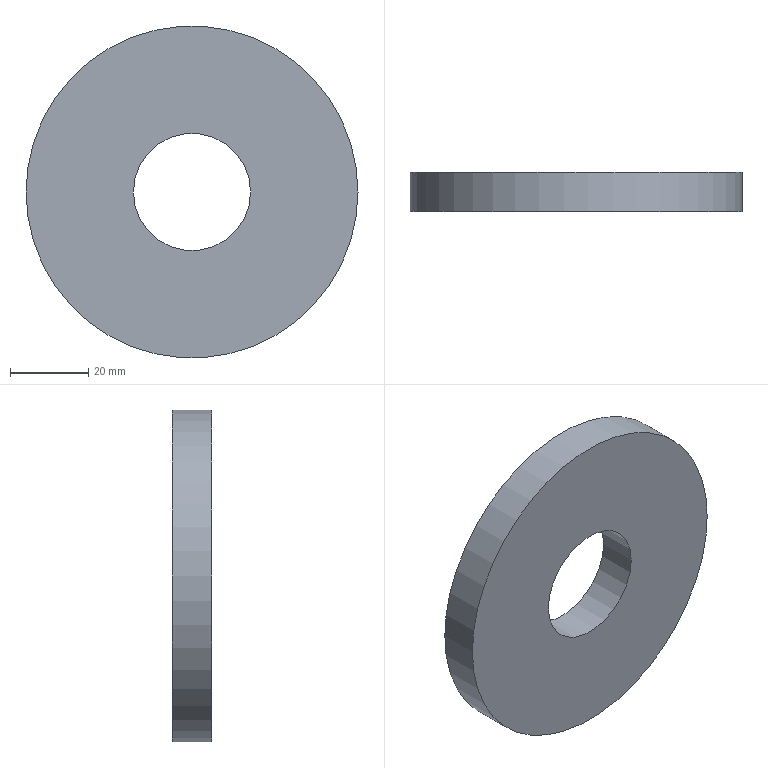Component | NX | SWASH_PLATE | 1 solid | 4 faces | box 85 x 10 x 85 mm | volume 49676 mm3 | cylinder 2 | plane 2 | commonest cylinder face diameters 85 x1 30 x1
STEP:
#1=CARTESIAN_POINT('',(0.,0.,0.));
#2=DIRECTION('',(0.,0.,1.));
#3=DIRECTION('',(1.,0.,0.));
#4=AXIS2_PLACEMENT_3D('',#1,#2,#3);
#5=CARTESIAN_POINT('',(42.5,99.,-0.));
#6=VERTEX_POINT('',#5);
#7=CARTESIAN_POINT('',(0.,99.,-0.));
#8=DIRECTION('',(0.,-1.,0.));
#9=DIRECTION('',(1.,0.,-0.));
#10=AXIS2_PLACEMENT_3D('',#7,#8,#9);
#11=CIRCLE('',#10,42.5);
#12=CARTESIAN_POINT('',(0.,99.,-0.));
#13=DIRECTION('',(0.,1.,0.));
#14=DIRECTION('',(0.,0.,1.));
#15=AXIS2_PLACEMENT_3D('',#12,#13,#14);
#16=CYLINDRICAL_SURFACE('',#15,42.5);
#17=CARTESIAN_POINT('',(7.854,0.));
#18=DIRECTION('',(-1.,0.));
#19=VECTOR('',#18,1.);
#20=LINE('',#17,#19);
#21=(GEOMETRIC_REPRESENTATION_CONTEXT(2)PARAMETRIC_REPRESENTATION_CONTEXT()REPRESENTATION_CONTEXT('',''));
#22=DEFINITIONAL_REPRESENTATION('',(#20),#21);
#23=PCURVE('',#16,#22);
#24=CARTESIAN_POINT('',(0.,99.,-0.));
#25=DIRECTION('',(0.,-1.,0.));
#26=DIRECTION('',(0.,0.,-1.));
#27=AXIS2_PLACEMENT_3D('',#24,#25,#26);
#28=PLANE('',#27);
#29=CARTESIAN_POINT('',(0.,0.));
#30=DIRECTION('',(0.,1.));
#31=AXIS2_PLACEMENT_2D('',#29,#30);
#32=CIRCLE('',#31,42.5);
#33=(GEOMETRIC_REPRESENTATION_CONTEXT(2)PARAMETRIC_REPRESENTATION_CONTEXT()REPRESENTATION_CONTEXT('',''));
#34=DEFINITIONAL_REPRESENTATION('',(#32),#33);
#35=PCURVE('',#28,#34);
#36=SURFACE_CURVE('',#11,(#23,#35),.PCURVE_S1.);
#37=EDGE_CURVE('',#6,#6,#36,.T.);
#38=ORIENTED_EDGE('',*,*,#37,.F.);
#39=CARTESIAN_POINT('',(42.5,109.,-0.));
#40=VERTEX_POINT('',#39);
#41=CARTESIAN_POINT('',(42.5,99.,-0.));
#42=CARTESIAN_POINT('',(42.5,109.,-0.));
#43=B_SPLINE_CURVE_WITH_KNOTS('',1,(#41,#42),.UNSPECIFIED.,.F.,.F.,(2,2),(0.,10.),.PIECEWISE_BEZIER_KNOTS.);
#44=CARTESIAN_POINT('',(7.854,0.));
#45=DIRECTION('',(0.,1.));
#46=VECTOR('',#45,1.);
#47=LINE('',#44,#46);
#48=(GEOMETRIC_REPRESENTATION_CONTEXT(2)PARAMETRIC_REPRESENTATION_CONTEXT()REPRESENTATION_CONTEXT('',''));
#49=DEFINITIONAL_REPRESENTATION('',(#47),#48);
#50=PCURVE('',#16,#49);
#51=CARTESIAN_POINT('',(1.571,0.));
#52=DIRECTION('',(0.,1.));
#53=VECTOR('',#52,1.);
#54=LINE('',#51,#53);
#55=(GEOMETRIC_REPRESENTATION_CONTEXT(2)PARAMETRIC_REPRESENTATION_CONTEXT()REPRESENTATION_CONTEXT('',''));
#56=DEFINITIONAL_REPRESENTATION('',(#54),#55);
#57=PCURVE('',#16,#56);
#58=SEAM_CURVE('',#43,(#50,#57),.PCURVE_S1.);
#59=EDGE_CURVE('',#6,#40,#58,.T.);
#60=ORIENTED_EDGE('',*,*,#59,.T.);
#61=CARTESIAN_POINT('',(0.,109.,-0.));
#62=DIRECTION('',(0.,-1.,0.));
#63=DIRECTION('',(1.,0.,-0.));
#64=AXIS2_PLACEMENT_3D('',#61,#62,#63);
#65=CIRCLE('',#64,42.5);
#66=CARTESIAN_POINT('',(7.854,10.));
#67=DIRECTION('',(-1.,0.));
#68=VECTOR('',#67,1.);
#69=LINE('',#66,#68);
#70=(GEOMETRIC_REPRESENTATION_CONTEXT(2)PARAMETRIC_REPRESENTATION_CONTEXT()REPRESENTATION_CONTEXT('',''));
#71=DEFINITIONAL_REPRESENTATION('',(#69),#70);
#72=PCURVE('',#16,#71);
#73=CARTESIAN_POINT('',(0.,109.,-0.));
#74=DIRECTION('',(0.,-1.,0.));
#75=DIRECTION('',(0.,0.,-1.));
#76=AXIS2_PLACEMENT_3D('',#73,#74,#75);
#77=PLANE('',#76);
#78=CARTESIAN_POINT('',(0.,0.));
#79=DIRECTION('',(0.,1.));
#80=AXIS2_PLACEMENT_2D('',#78,#79);
#81=CIRCLE('',#80,42.5);
#82=(GEOMETRIC_REPRESENTATION_CONTEXT(2)PARAMETRIC_REPRESENTATION_CONTEXT()REPRESENTATION_CONTEXT('',''));
#83=DEFINITIONAL_REPRESENTATION('',(#81),#82);
#84=PCURVE('',#77,#83);
#85=SURFACE_CURVE('',#65,(#72,#84),.PCURVE_S1.);
#86=EDGE_CURVE('',#40,#40,#85,.T.);
#87=ORIENTED_EDGE('',*,*,#86,.T.);
#88=ORIENTED_EDGE('',*,*,#59,.F.);
#89=EDGE_LOOP('',(#38,#60,#87,#88));
#90=FACE_BOUND('',#89,.T.);
#91=ADVANCED_FACE('',(#90),#16,.T.);
#92=CARTESIAN_POINT('',(15.,99.,-0.));
#93=VERTEX_POINT('',#92);
#94=CARTESIAN_POINT('',(0.,99.,-0.));
#95=DIRECTION('',(0.,-1.,0.));
#96=DIRECTION('',(1.,0.,-0.));
#97=AXIS2_PLACEMENT_3D('',#94,#95,#96);
#98=CIRCLE('',#97,15.);
#99=CARTESIAN_POINT('',(0.,99.,-0.));
#100=DIRECTION('',(0.,1.,0.));
#101=DIRECTION('',(0.,0.,1.));
#102=AXIS2_PLACEMENT_3D('',#99,#100,#101);
#103=CYLINDRICAL_SURFACE('',#102,15.);
#104=CARTESIAN_POINT('',(7.854,0.));
#105=DIRECTION('',(-1.,0.));
#106=VECTOR('',#105,1.);
#107=LINE('',#104,#106);
#108=(GEOMETRIC_REPRESENTATION_CONTEXT(2)PARAMETRIC_REPRESENTATION_CONTEXT()REPRESENTATION_CONTEXT('',''));
#109=DEFINITIONAL_REPRESENTATION('',(#107),#108);
#110=PCURVE('',#103,#109);
#111=CARTESIAN_POINT('',(0.,0.));
#112=DIRECTION('',(0.,1.));
#113=AXIS2_PLACEMENT_2D('',#111,#112);
#114=CIRCLE('',#113,15.);
#115=(GEOMETRIC_REPRESENTATION_CONTEXT(2)PARAMETRIC_REPRESENTATION_CONTEXT()REPRESENTATION_CONTEXT('',''));
#116=DEFINITIONAL_REPRESENTATION('',(#114),#115);
#117=PCURVE('',#28,#116);
#118=SURFACE_CURVE('',#98,(#110,#117),.PCURVE_S1.);
#119=EDGE_CURVE('',#93,#93,#118,.T.);
#120=ORIENTED_EDGE('',*,*,#119,.F.);
#121=CARTESIAN_POINT('',(15.,109.,-0.));
#122=VERTEX_POINT('',#121);
#123=CARTESIAN_POINT('',(15.,99.,-0.));
#124=CARTESIAN_POINT('',(15.,109.,-0.));
#125=B_SPLINE_CURVE_WITH_KNOTS('',1,(#123,#124),.UNSPECIFIED.,.F.,.F.,(2,2),(0.,10.),.PIECEWISE_BEZIER_KNOTS.);
#126=CARTESIAN_POINT('',(7.854,0.));
#127=DIRECTION('',(0.,1.));
#128=VECTOR('',#127,1.);
#129=LINE('',#126,#128);
#130=(GEOMETRIC_REPRESENTATION_CONTEXT(2)PARAMETRIC_REPRESENTATION_CONTEXT()REPRESENTATION_CONTEXT('',''));
#131=DEFINITIONAL_REPRESENTATION('',(#129),#130);
#132=PCURVE('',#103,#131);
#133=CARTESIAN_POINT('',(1.571,0.));
#134=DIRECTION('',(0.,1.));
#135=VECTOR('',#134,1.);
#136=LINE('',#133,#135);
#137=(GEOMETRIC_REPRESENTATION_CONTEXT(2)PARAMETRIC_REPRESENTATION_CONTEXT()REPRESENTATION_CONTEXT('',''));
#138=DEFINITIONAL_REPRESENTATION('',(#136),#137);
#139=PCURVE('',#103,#138);
#140=SEAM_CURVE('',#125,(#132,#139),.PCURVE_S1.);
#141=EDGE_CURVE('',#93,#122,#140,.T.);
#142=ORIENTED_EDGE('',*,*,#141,.T.);
#143=CARTESIAN_POINT('',(0.,109.,-0.));
#144=DIRECTION('',(0.,-1.,0.));
#145=DIRECTION('',(1.,0.,-0.));
#146=AXIS2_PLACEMENT_3D('',#143,#144,#145);
#147=CIRCLE('',#146,15.);
#148=CARTESIAN_POINT('',(7.854,10.));
#149=DIRECTION('',(-1.,0.));
#150=VECTOR('',#149,1.);
#151=LINE('',#148,#150);
#152=(GEOMETRIC_REPRESENTATION_CONTEXT(2)PARAMETRIC_REPRESENTATION_CONTEXT()REPRESENTATION_CONTEXT('',''));
#153=DEFINITIONAL_REPRESENTATION('',(#151),#152);
#154=PCURVE('',#103,#153);
#155=CARTESIAN_POINT('',(0.,0.));
#156=DIRECTION('',(0.,1.));
#157=AXIS2_PLACEMENT_2D('',#155,#156);
#158=CIRCLE('',#157,15.);
#159=(GEOMETRIC_REPRESENTATION_CONTEXT(2)PARAMETRIC_REPRESENTATION_CONTEXT()REPRESENTATION_CONTEXT('',''));
#160=DEFINITIONAL_REPRESENTATION('',(#158),#159);
#161=PCURVE('',#77,#160);
#162=SURFACE_CURVE('',#147,(#154,#161),.PCURVE_S1.);
#163=EDGE_CURVE('',#122,#122,#162,.T.);
#164=ORIENTED_EDGE('',*,*,#163,.T.);
#165=ORIENTED_EDGE('',*,*,#141,.F.);
#166=EDGE_LOOP('',(#120,#142,#164,#165));
#167=FACE_BOUND('',#166,.F.);
#168=ADVANCED_FACE('',(#167),#103,.F.);
#169=ORIENTED_EDGE('',*,*,#37,.T.);
#170=EDGE_LOOP('',(#169));
#171=FACE_BOUND('',#170,.T.);
#172=ORIENTED_EDGE('',*,*,#119,.F.);
#173=EDGE_LOOP('',(#172));
#174=FACE_BOUND('',#173,.T.);
#175=ADVANCED_FACE('',(#171,#174),#28,.T.);
#176=ORIENTED_EDGE('',*,*,#86,.F.);
#177=EDGE_LOOP('',(#176));
#178=FACE_BOUND('',#177,.T.);
#179=ORIENTED_EDGE('',*,*,#163,.T.);
#180=EDGE_LOOP('',(#179));
#181=FACE_BOUND('',#180,.T.);
#182=ADVANCED_FACE('',(#178,#181),#77,.F.);
#183=CLOSED_SHELL('',(#91,#168,#175,#182));
#184=MANIFOLD_SOLID_BREP('',#183);
#185=(LENGTH_UNIT()NAMED_UNIT(*)SI_UNIT(.MILLI.,.METRE.));
#186=UNCERTAINTY_MEASURE_WITH_UNIT(LENGTH_MEASURE(0.00001),#185,'','');
#187=(NAMED_UNIT(*)PLANE_ANGLE_UNIT()SI_UNIT($,.RADIAN.));
#188=(NAMED_UNIT(*)SI_UNIT($,.STERADIAN.)SOLID_ANGLE_UNIT());
#189=(GEOMETRIC_REPRESENTATION_CONTEXT(3)GLOBAL_UNCERTAINTY_ASSIGNED_CONTEXT((#186))GLOBAL_UNIT_ASSIGNED_CONTEXT((#185,#187,#188))REPRESENTATION_CONTEXT('',''));
#190=ADVANCED_BREP_SHAPE_REPRESENTATION('',(#4,#184),#189);